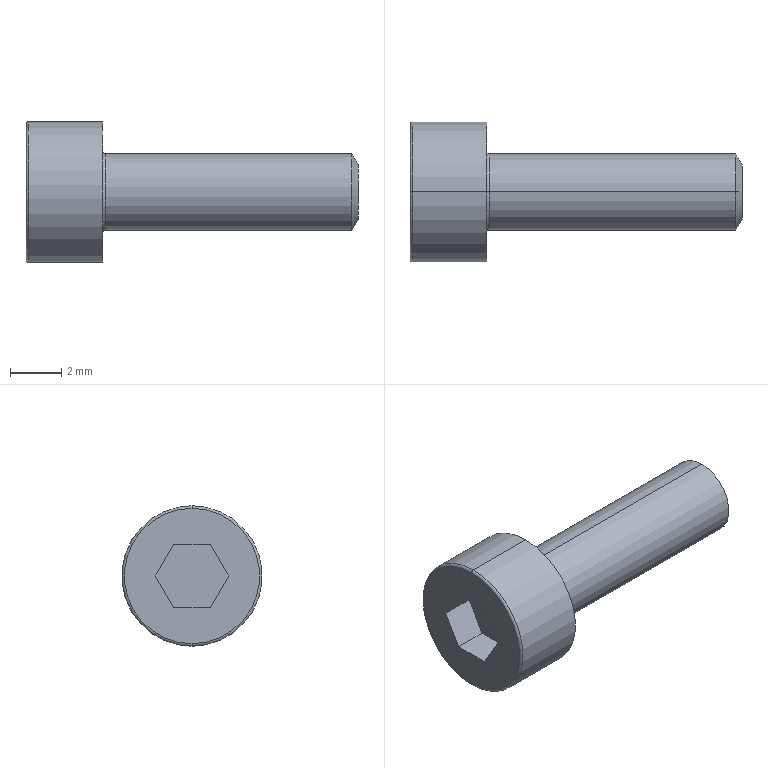Component | NX | HEX_SOCKET_CAP_SCREW_M3X10_3 | 1 solid | 20 faces | volume 135 mm3 | plane 10 | torus 4 | cylinder 4 | cone 2 | commonest cylinder face diameters 5.5 x2 3 x2